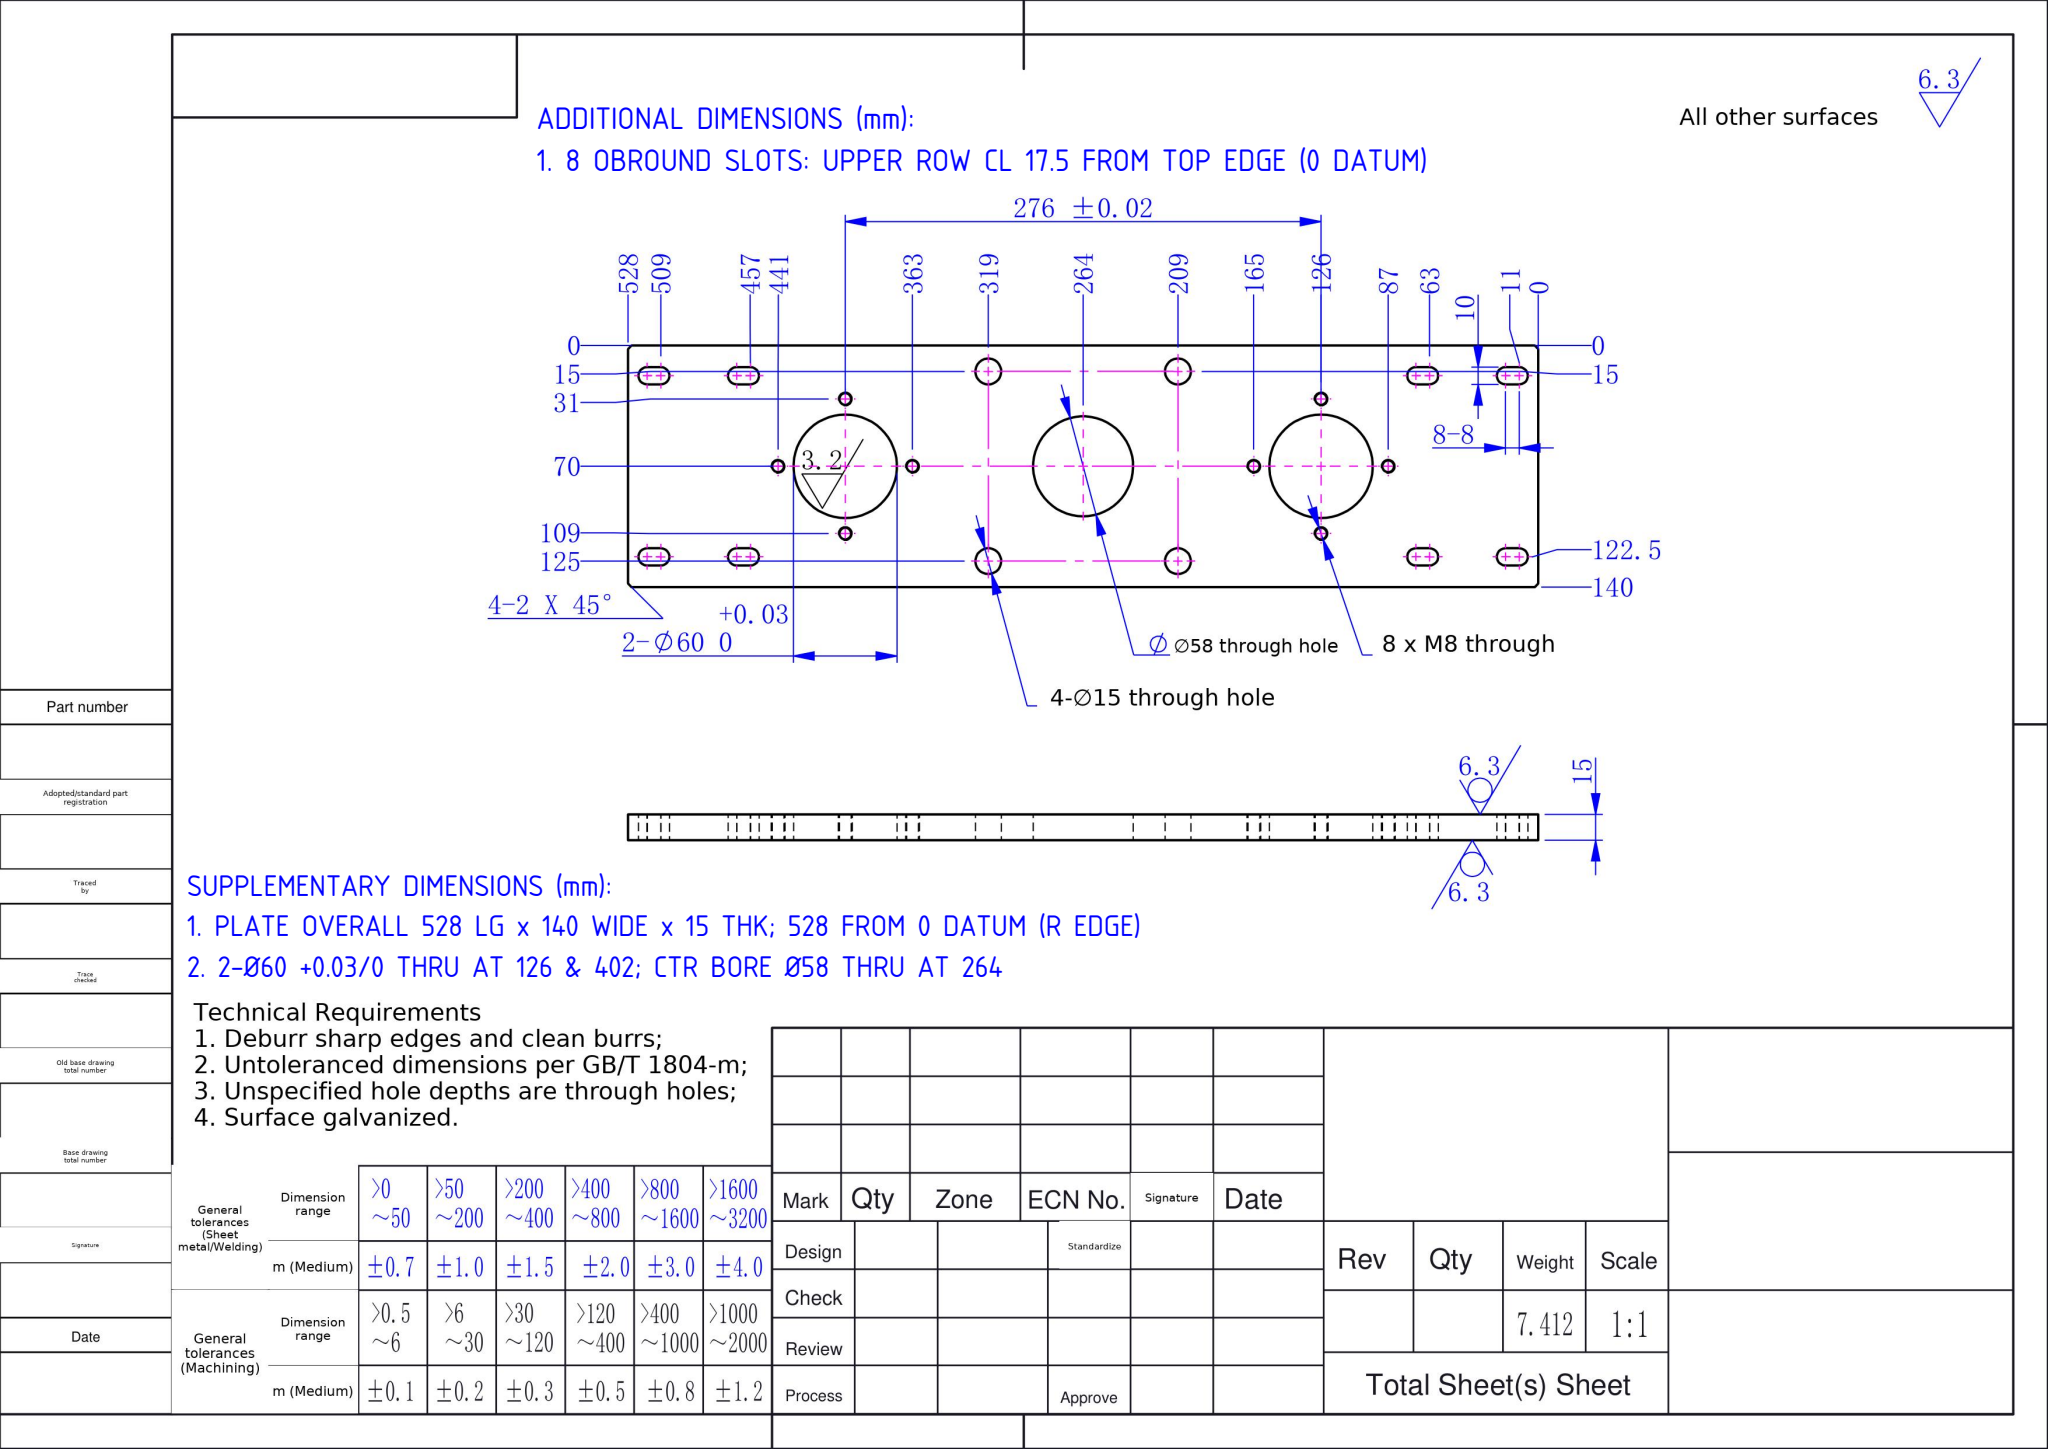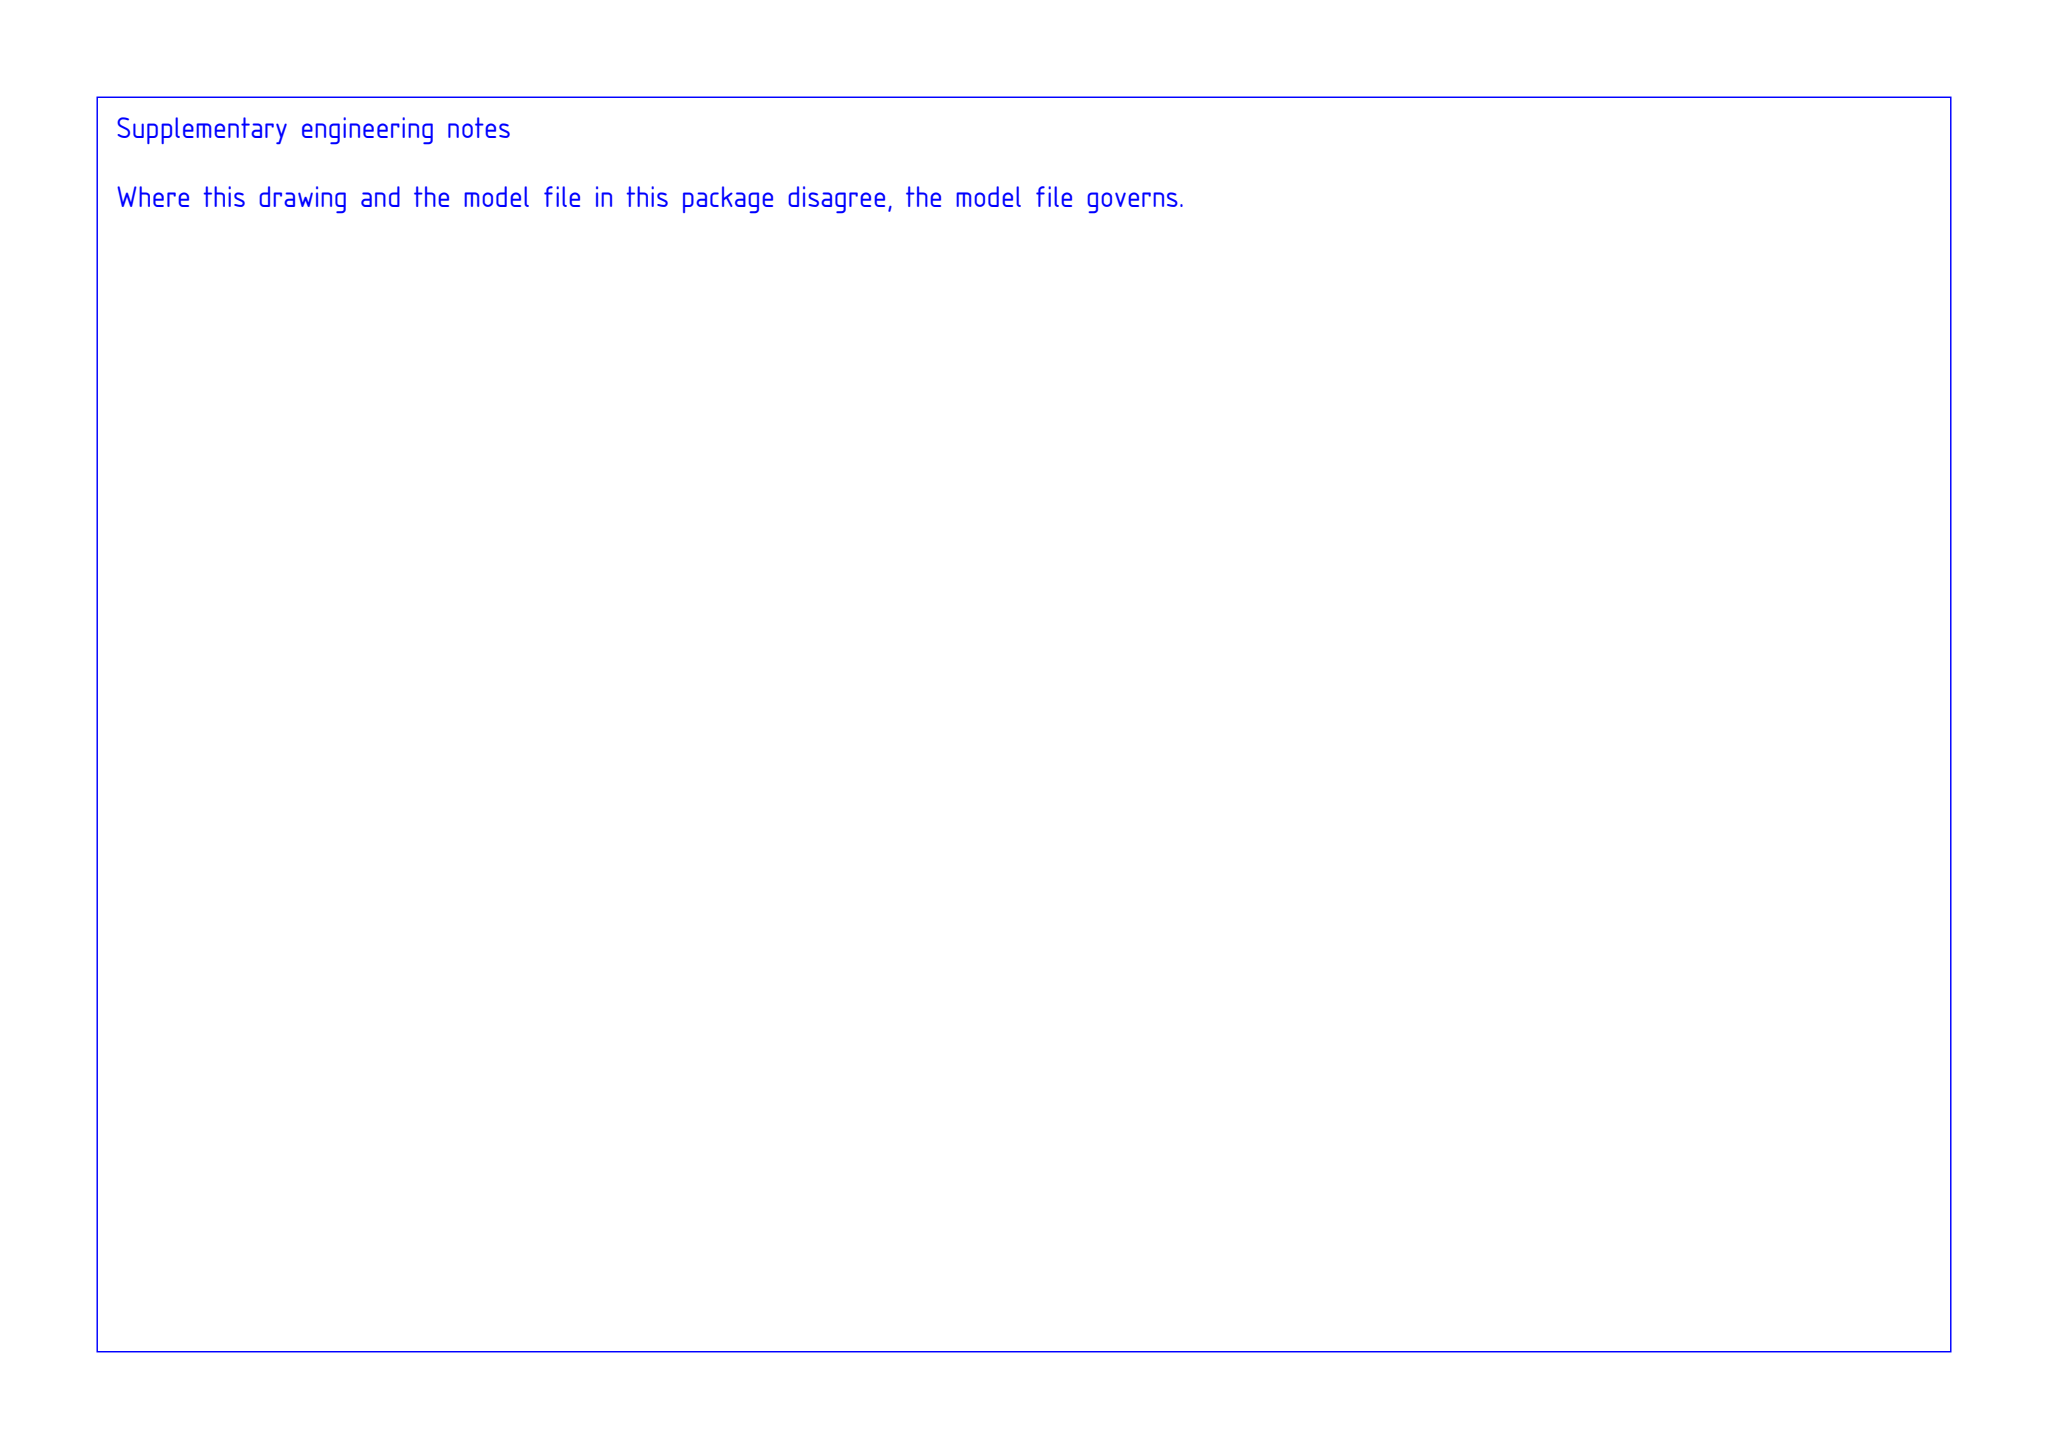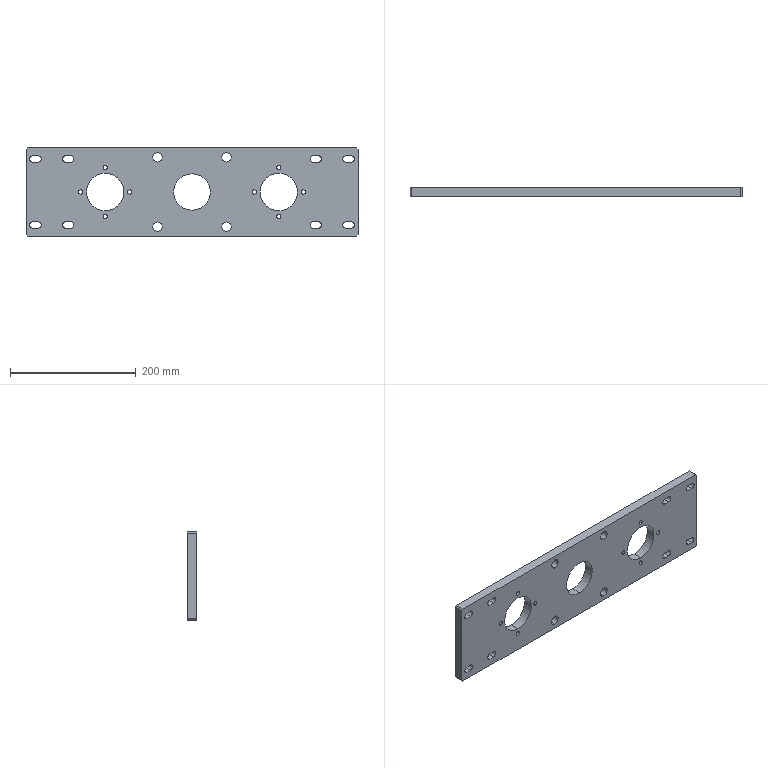Part | SolidWorks | mm | 1 solid | 72 faces | box 528 x 15 x 140 mm | volume 950240 mm3 | cylinder 46 | plane 26 | commonest cylinder face diameters 6.8 x16 10 x16 15 x8 60 x4 58 x2
build123d program:
from build123d import *

# Parameters (mm, degrees)
SKETCH1_W           = 528
SKETCH1_H           = 140
BOSS_EXTRUDE1_DEPTH = 15
CHAMFER1_SIZE       = 2
CUT_EXTRUDE1_REACH  = 275.534
CUT_EXTRUDE2_REACH  = 275.534
SKETCH3_R           = 29
SKETCH3_R_2         = 30
M8_TAPPED_HOLE1_D   = 6.8
SKETCH6_R           = 7.5
CUT_EXTRUDE3_DEPTH  = 22


with BuildPart() as part:
    # Sketch1 → Boss-Extrude1 (new body)
    with BuildSketch(Plane(origin=(0, 0, 0), x_dir=(1, 0, 0), z_dir=(0, 1, 0))):
        Rectangle(SKETCH1_W, SKETCH1_H)
    extrude(amount=BOSS_EXTRUDE1_DEPTH)

    # Chamfer1
    chamfer1_edges = [part.edges().sort_by_distance(p)[0] for p in [
        (264, 7.5, 70),
        (-264, 7.5, 70),
        (-264, 7.5, -70),
        (264, 7.5, -70),
    ]]
    chamfer(chamfer1_edges, length=CHAMFER1_SIZE)

    # Sketch2 → Cut-Extrude1 (cut, up to next)
    with BuildSketch(Plane(origin=(0, 15, 0), x_dir=(1, 0, 0), z_dir=(0, 1, 0)), mode=Mode.PRIVATE) as cut_extrude1_sk1:
        with BuildLine():
            Line((-253, 57.5), (-245, 57.5))
            ThreePointArc((-245, 57.5), (-240, 52.5), (-245, 47.5))
            Line((-245, 47.5), (-253, 47.5))
            ThreePointArc((-253, 47.5), (-258, 52.5), (-253, 57.5))
        make_face()
    cut_extrude1_tool1 = extrude(cut_extrude1_sk1.sketch, amount=-CUT_EXTRUDE1_REACH, mode=Mode.PRIVATE) & part.part
    # Sketch2 → Cut-Extrude1 (cut, up to next)
    with BuildSketch(Plane(origin=(0, 15, 0), x_dir=(1, 0, 0), z_dir=(0, 1, 0)), mode=Mode.PRIVATE) as cut_extrude1_sk2:
        with BuildLine():
            Line((-253, -47.5), (-245, -47.5))
            ThreePointArc((-245, -47.5), (-240, -52.5), (-245, -57.5))
            Line((-245, -57.5), (-253, -57.5))
            ThreePointArc((-253, -57.5), (-258, -52.5), (-253, -47.5))
        make_face()
    cut_extrude1_tool2 = extrude(cut_extrude1_sk2.sketch, amount=-CUT_EXTRUDE1_REACH, mode=Mode.PRIVATE) & part.part
    # Sketch2 → Cut-Extrude1 (cut, up to next)
    with BuildSketch(Plane(origin=(0, 15, 0), x_dir=(1, 0, 0), z_dir=(0, 1, 0)), mode=Mode.PRIVATE) as cut_extrude1_sk3:
        with BuildLine():
            Line((-201, 57.5), (-193, 57.5))
            ThreePointArc((-193, 57.5), (-188, 52.5), (-193, 47.5))
            Line((-193, 47.5), (-201, 47.5))
            ThreePointArc((-201, 47.5), (-206, 52.5), (-201, 57.5))
        make_face()
    cut_extrude1_tool3 = extrude(cut_extrude1_sk3.sketch, amount=-CUT_EXTRUDE1_REACH, mode=Mode.PRIVATE) & part.part
    # Sketch2 → Cut-Extrude1 (cut, up to next)
    with BuildSketch(Plane(origin=(0, 15, 0), x_dir=(1, 0, 0), z_dir=(0, 1, 0)), mode=Mode.PRIVATE) as cut_extrude1_sk4:
        with BuildLine():
            Line((-201, -47.5), (-193, -47.5))
            ThreePointArc((-193, -47.5), (-188, -52.5), (-193, -57.5))
            Line((-193, -57.5), (-201, -57.5))
            ThreePointArc((-201, -57.5), (-206, -52.5), (-201, -47.5))
        make_face()
    cut_extrude1_tool4 = extrude(cut_extrude1_sk4.sketch, amount=-CUT_EXTRUDE1_REACH, mode=Mode.PRIVATE) & part.part
    cut_extrude1_1 = cut_extrude1_tool1.solids().sort_by_distance((-249, 15, -52.5))[0]
    add(cut_extrude1_1, mode=Mode.SUBTRACT)
    cut_extrude1_2 = cut_extrude1_tool2.solids().sort_by_distance((-249, 15, 52.5))[0]
    add(cut_extrude1_2, mode=Mode.SUBTRACT)
    cut_extrude1_3 = cut_extrude1_tool3.solids().sort_by_distance((-197, 15, -52.5))[0]
    add(cut_extrude1_3, mode=Mode.SUBTRACT)
    cut_extrude1_4 = cut_extrude1_tool4.solids().sort_by_distance((-197, 15, 52.5))[0]
    add(cut_extrude1_4, mode=Mode.SUBTRACT)
    cut_extrude1 = cut_extrude1_1 + cut_extrude1_2 + cut_extrude1_3 + cut_extrude1_4  # Cut-Extrude1 as one shape, for the pattern or mirror that repeats it

    # Sketch3 → Cut-Extrude2 (cut, up to next)
    with BuildSketch(Plane(origin=(0, 15, 0), x_dir=(1, 0, 0), z_dir=(0, 1, 0)), mode=Mode.PRIVATE) as cut_extrude2_sk1:
        with Locations(Location((0, 0, 0), (0, 0, 270))):
            Circle(SKETCH3_R)
    cut_extrude2_tool1 = extrude(cut_extrude2_sk1.sketch, amount=-CUT_EXTRUDE2_REACH, mode=Mode.PRIVATE) & part.part
    # Sketch3 → Cut-Extrude2 (cut, up to next)
    with BuildSketch(Plane(origin=(0, 15, 0), x_dir=(1, 0, 0), z_dir=(0, 1, 0)), mode=Mode.PRIVATE) as cut_extrude2_sk2:
        with Locations(Location((-138, 0, 0), (0, 0, 270))):
            Circle(SKETCH3_R_2)
    cut_extrude2_tool2 = extrude(cut_extrude2_sk2.sketch, amount=-CUT_EXTRUDE2_REACH, mode=Mode.PRIVATE) & part.part
    # Sketch3 → Cut-Extrude2 (cut, up to next)
    with BuildSketch(Plane(origin=(0, 15, 0), x_dir=(1, 0, 0), z_dir=(0, 1, 0)), mode=Mode.PRIVATE) as cut_extrude2_sk3:
        with Locations(Location((138, 0, 0), (0, 0, 270))):
            Circle(SKETCH3_R_2)
    cut_extrude2_tool3 = extrude(cut_extrude2_sk3.sketch, amount=-CUT_EXTRUDE2_REACH, mode=Mode.PRIVATE) & part.part
    add(cut_extrude2_tool1.solids().sort_by_distance((0, 15, 0))[0], mode=Mode.SUBTRACT)
    add(cut_extrude2_tool2.solids().sort_by_distance((-138, 15, 0))[0], mode=Mode.SUBTRACT)
    add(cut_extrude2_tool3.solids().sort_by_distance((138, 15, 0))[0], mode=Mode.SUBTRACT)

    # M8 Tapped Hole1 (through all)
    with Locations(Plane(origin=(0, 15, 0), x_dir=(1, 0, 0), z_dir=(0, 1, 0))):
        with Locations((-138, 39), (-138, -39), (-177, 0), (-99, 0)):
            m8_tapped_hole1 = Hole(M8_TAPPED_HOLE1_D / 2)

    # Mirror1: M8 Tapped Hole1 across plane
    add(m8_tapped_hole1.mirror(Plane(origin=(0, 0, 0), x_dir=(0, 0, 1), z_dir=(1, 0, 0))), mode=Mode.SUBTRACT)

    # Sketch6 → Cut-Extrude3 (cut)
    with BuildSketch(Plane(origin=(0, 15, 0), x_dir=(1, 0, 0), z_dir=(0, 1, 0))):
        with Locations(Location((-55, 55, 0), (0, 0, 270))):
            Circle(SKETCH6_R)
        with Locations(Location((55, 55, 0), (0, 0, 270))):
            Circle(SKETCH6_R)
        with Locations(Location((55, -55, 0), (0, 0, 270))):
            Circle(SKETCH6_R)
        with Locations(Location((-55, -55, 0), (0, 0, 270))):
            Circle(SKETCH6_R)
    extrude(amount=-CUT_EXTRUDE3_DEPTH, mode=Mode.SUBTRACT)

    # Mirror2: Cut-Extrude1 across plane
    add(cut_extrude1.mirror(Plane(origin=(0, 0, 0), x_dir=(0, 0, 1), z_dir=(1, 0, 0))), mode=Mode.SUBTRACT)


solid = part.part